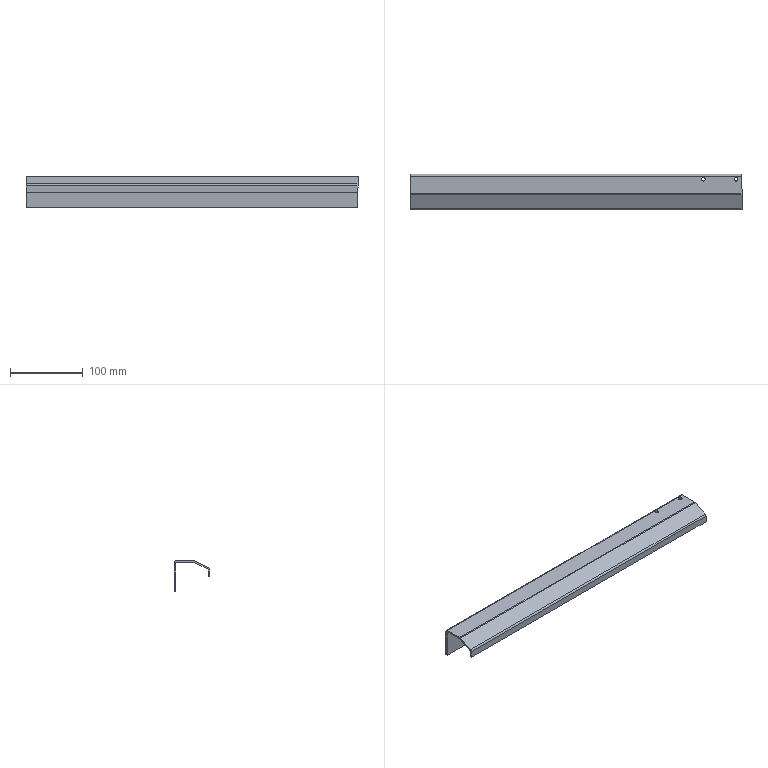Component | SolidWorks | DrawerAssembly-1_Handle-1 | 1 solid | 46 faces | volume 90338 mm3 | plane 30 | cylinder 16 | commonest cylinder face diameters 7 x6 5 x4 2 x3 6 x3